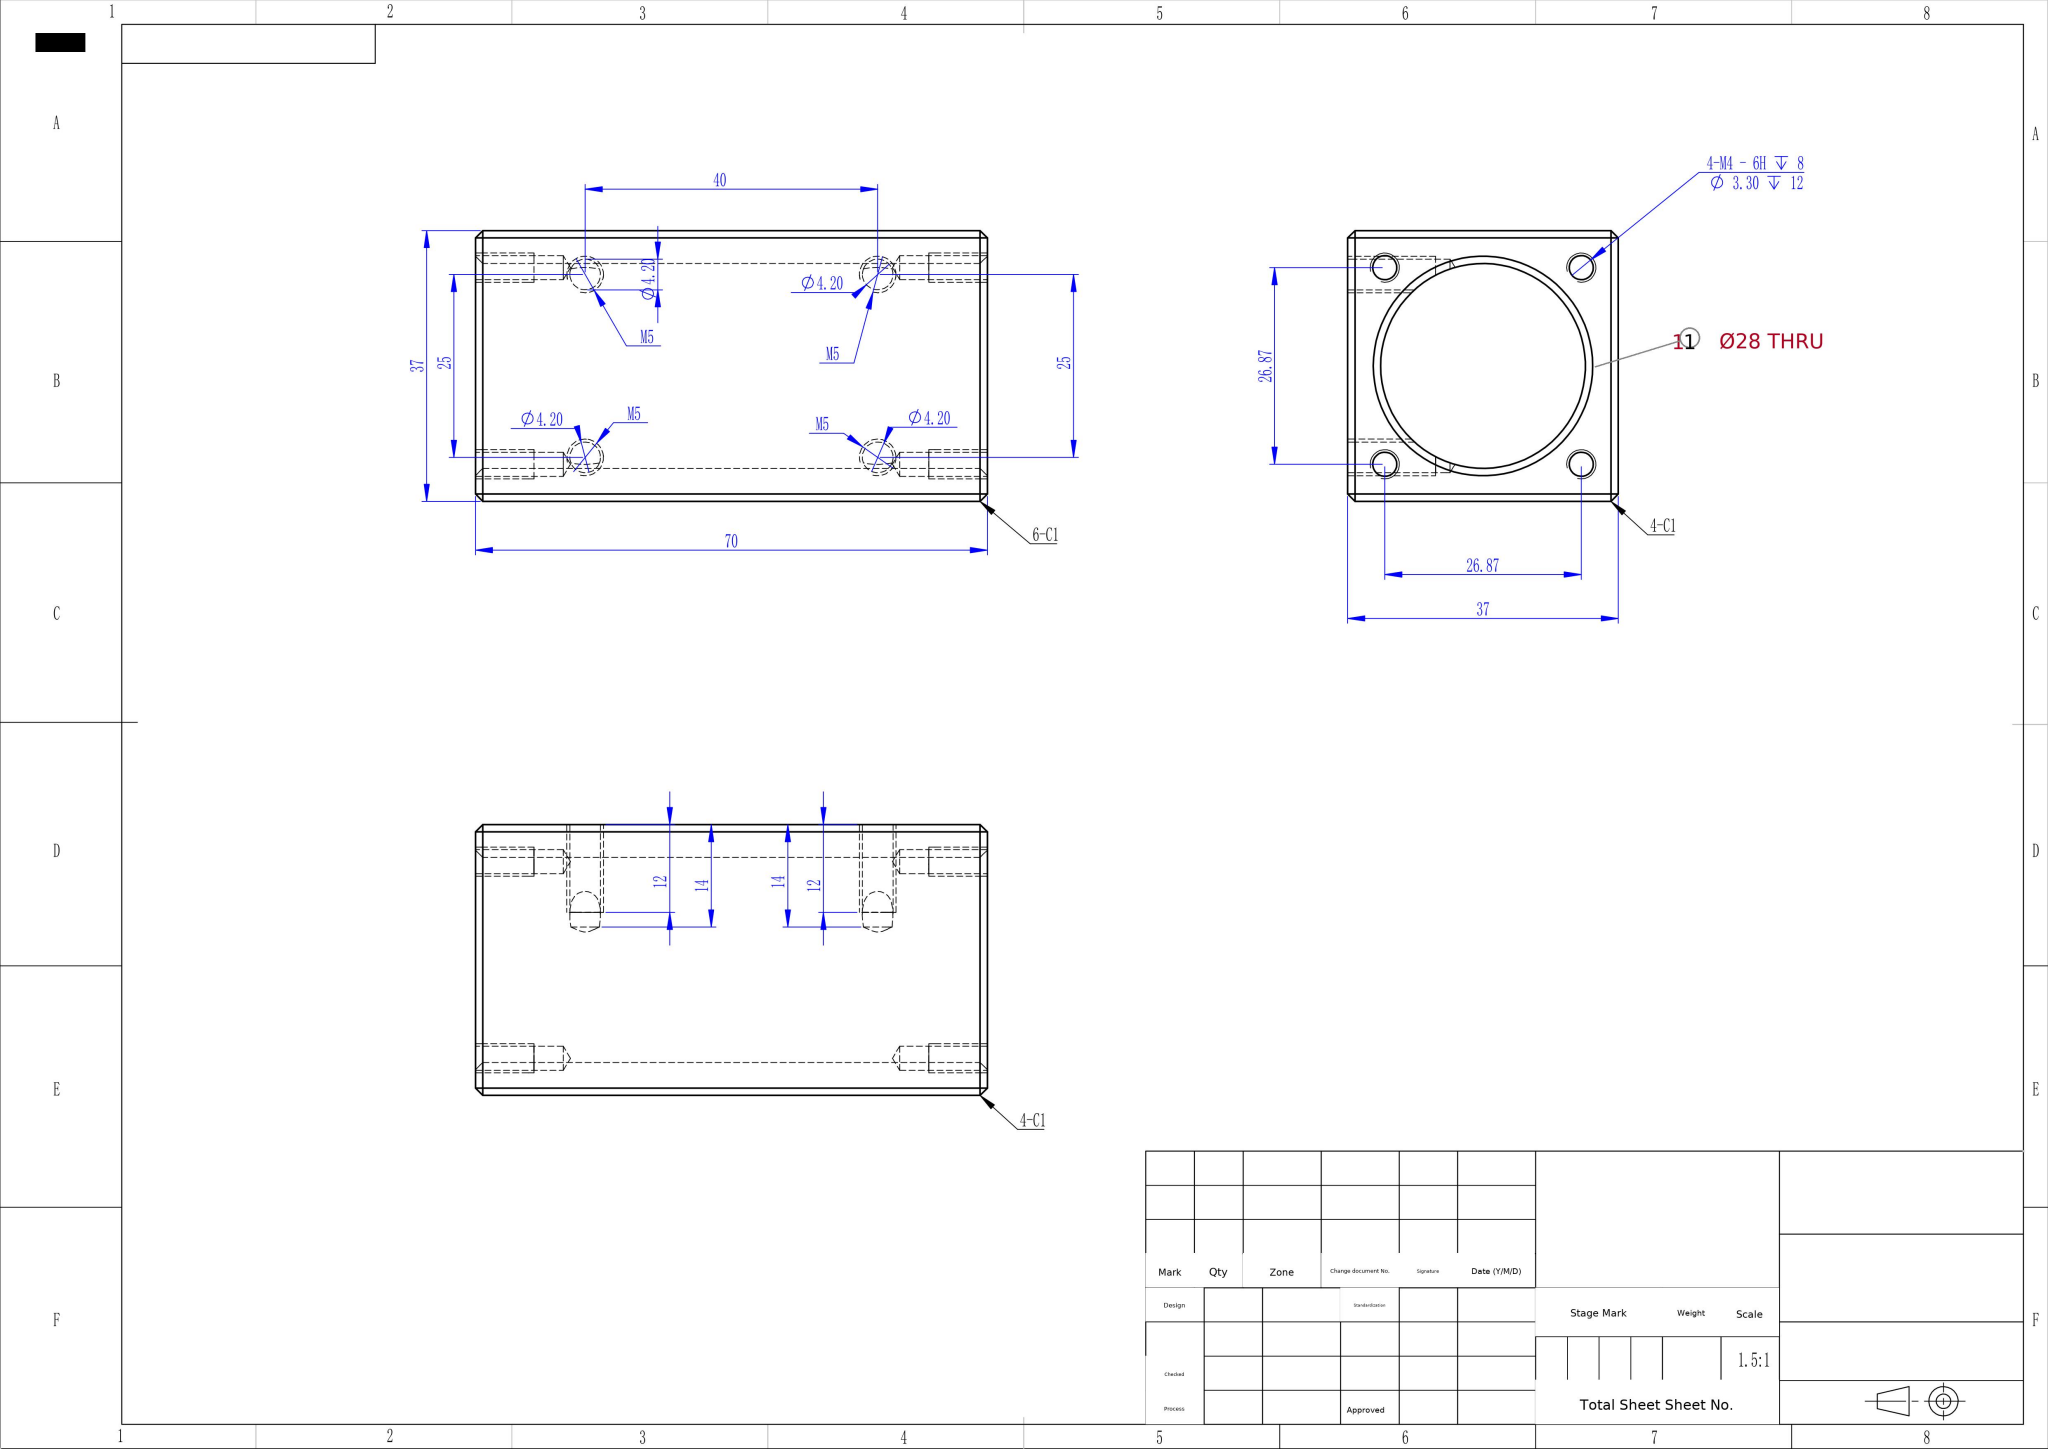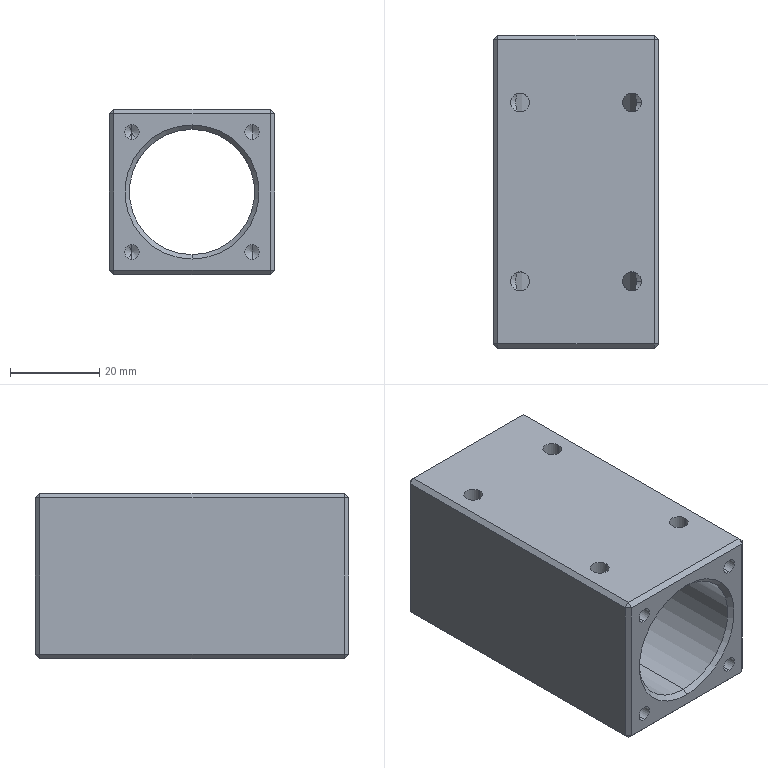Part | SolidWorks | mm | 1 solid | 78 faces | box 37 x 70 x 37 mm | volume 50834 mm3 | cone 26 | cylinder 26 | plane 26 | commonest cylinder face diameters 3.3 x16 4.2 x8 28 x2
build123d program:
from build123d import *

# Parameters (mm, degrees)
SKETCH1_W                  = 37
SKETCH1_H                  = 70
BOSS_EXTRUDE1_DEPTH        = 18.5
SKETCH2_R                  = 14
CUT_EXTRUDE1_DEPTH         = 75.73
M4_TAPPED_HOLE1_AT_2_COUNT = 2
M4_TAPPED_HOLE1_AT_2_PITCH = 26.87
M4_TAPPED_HOLE1_AT_3_COUNT = 2
M4_TAPPED_HOLE1_AT_3_PITCH = 38
M4_TAPPED_HOLE1_AT_4_COUNT = 2
M4_TAPPED_HOLE1_AT_4_PITCH = 26.87
M5_TAPPED_HOLE1_D          = 4.2
M5_TAPPED_HOLE1_DEPTH      = 14
M5_TAPPED_HOLE1_TIP        = 1.262
CHAMFER1_SIZE              = 1


with BuildPart() as part:
    # Sketch1 → Boss-Extrude1 (new, symmetric)
    with BuildSketch(Plane.XY):
        Rectangle(SKETCH1_W, SKETCH1_H)
    extrude(amount=BOSS_EXTRUDE1_DEPTH, both=True)

    # Sketch2 → Cut-Extrude1 (cut, through all)
    with BuildSketch(Plane(origin=(0, 35, 0), x_dir=(1, 0, 0), z_dir=(0, 1, 0))):
        with Locations(Location((0, 0, 0), (0, 0, 270))):
            Circle(SKETCH2_R)
    extrude(amount=-CUT_EXTRUDE1_DEPTH, mode=Mode.SUBTRACT)

    # Sketch5 → M4 Tapped Hole1 (revolve, cut)
    with BuildSketch(Plane(origin=(-13.435, 35, -13.435), x_dir=(0, 0, 1), z_dir=(1, 0, 0))):
        Polygon((0, 0), (0, 12.991), (1.65, 12), (1.65, 0), align=None)
    m4_tapped_hole1 = revolve(axis=Axis((-13.435, 41.35, -13.435), (0, -1, 0)), mode=Mode.SUBTRACT)

    # M4 Tapped Hole1 at 2: M4 Tapped Hole1 ×2
    with Locations(*[(0, 0, i * M4_TAPPED_HOLE1_AT_2_PITCH) for i in range(1, M4_TAPPED_HOLE1_AT_2_COUNT)]):
        add(m4_tapped_hole1, mode=Mode.SUBTRACT)

    # M4 Tapped Hole1 at 3: M4 Tapped Hole1 ×2
    with Locations(*[Vector(0.7071, 0, 0.7071) * (i * M4_TAPPED_HOLE1_AT_3_PITCH) for i in range(1, M4_TAPPED_HOLE1_AT_3_COUNT)]):
        add(m4_tapped_hole1, mode=Mode.SUBTRACT)

    # M4 Tapped Hole1 at 4: M4 Tapped Hole1 ×2
    with Locations(*[(i * M4_TAPPED_HOLE1_AT_4_PITCH, 0, 0) for i in range(1, M4_TAPPED_HOLE1_AT_4_COUNT)]):
        add(m4_tapped_hole1, mode=Mode.SUBTRACT)

    # Mirror1: M4 Tapped Hole1 across plane
    add(m4_tapped_hole1.mirror(Plane.ZX), mode=Mode.SUBTRACT)

    # Mirror1 copy 1 sketch → Mirror1 copy 1 (revolve, cut)
    with BuildSketch(Plane(origin=(-13.435, -35, 13.435), x_dir=(0, 0, 1), z_dir=(1, 0, 0))):
        Polygon((0, 0), (0, -12.991), (1.65, -12), (1.65, 0), align=None)
    revolve(axis=Axis((-13.435, -41.35, 13.435), (0, -1, 0)), mode=Mode.SUBTRACT)

    # Mirror1 copy 2 sketch → Mirror1 copy 2 (revolve, cut)
    with BuildSketch(Plane(origin=(13.435, -35, 13.435), x_dir=(0, 0, 1), z_dir=(1, 0, 0))):
        Polygon((0, 0), (0, -12.991), (1.65, -12), (1.65, 0), align=None)
    revolve(axis=Axis((13.435, -41.35, 13.435), (0, -1, 0)), mode=Mode.SUBTRACT)

    # Mirror1 copy 3 sketch → Mirror1 copy 3 (revolve, cut)
    with BuildSketch(Plane(origin=(13.435, -35, -13.435), x_dir=(0, 0, 1), z_dir=(1, 0, 0))):
        Polygon((0, 0), (0, -12.991), (1.65, -12), (1.65, 0), align=None)
    revolve(axis=Axis((13.435, -41.35, -13.435), (0, -1, 0)), mode=Mode.SUBTRACT)

    # M5 Tapped Hole1
    with Locations(Plane.XY.offset(18.5)):
        with Locations((-12.5, 20), (-12.5, -20), (12.5, -20), (12.5, 20)):
            Hole(M5_TAPPED_HOLE1_D / 2, depth=M5_TAPPED_HOLE1_DEPTH)
            with Locations((0, 0, -(M5_TAPPED_HOLE1_DEPTH + M5_TAPPED_HOLE1_TIP / 2))):  # 118° drill point
                Cone(0, M5_TAPPED_HOLE1_D / 2, M5_TAPPED_HOLE1_TIP, mode=Mode.SUBTRACT)

    # Chamfer1
    chamfer1_edges = [part.edges().sort_by_distance(p)[0] for p in [
        (-18.5, 0, 18.5),
        (0, -35, 18.5),
        (0, -35, -14),
        (0, 35, -14),
        (18.5, 0, 18.5),
        (0, -35, -18.5),
        (-18.5, 0, -18.5),
        (0, 35, -18.5),
        (18.5, 0, -18.5),
        (0, 35, 18.5),
        (18.5, -35, 0),
        (-18.5, -35, 0),
        (-18.5, 35, 0),
        (18.5, 35, 0),
    ]]
    chamfer(chamfer1_edges, length=CHAMFER1_SIZE)


solid = part.part